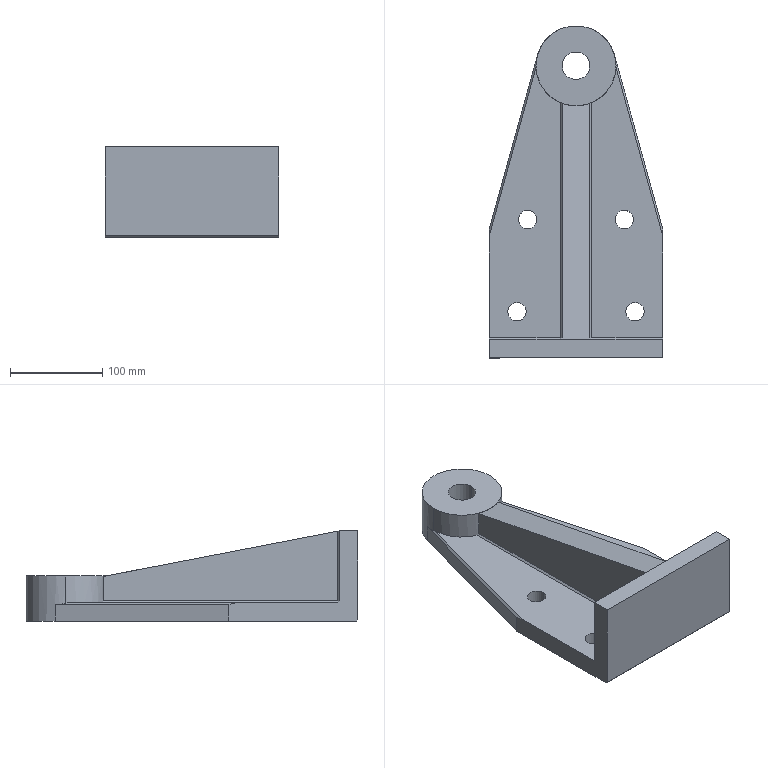Component | SolidWorks | SupportBase3-2 | 1 solid | 39 faces | volume 1891819 mm3 | plane 26 | cylinder 13 | commonest cylinder face diameters 20 x8 86.865 x3 30 x2 | material 45